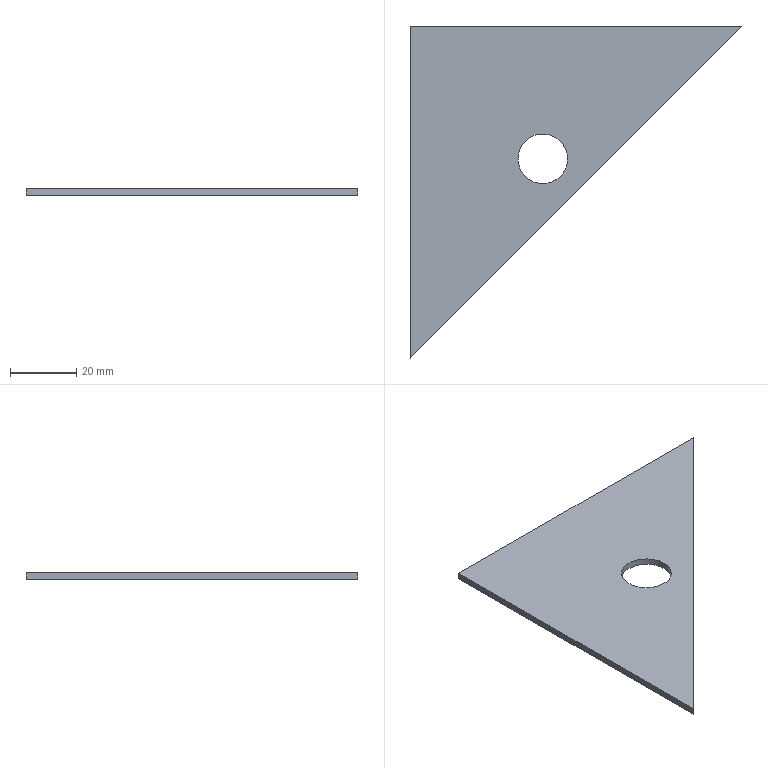Component | SolidWorks | GussetPlateAssembly-1_GussetPlate-1 | 1 solid | 7 faces | box 100 x 100 x 2 mm | volume 9647 mm3 | plane 5 | cylinder 2 | commonest cylinder face diameters 15 x2
STEP:
#1=CARTESIAN_POINT('',(-17.916,13.265,3.071));
#2=VERTEX_POINT('',#1);
#3=CARTESIAN_POINT('',(-17.326,13.265,3.071));
#4=VERTEX_POINT('',#3);
#5=CARTESIAN_POINT('',(-17.621,13.265,3.071));
#6=DIRECTION('',(0.,-0.,-1.));
#7=DIRECTION('',(1.,0.,0.));
#8=AXIS2_PLACEMENT_3D('',#5,#6,#7);
#9=CIRCLE('',#8,0.2953);
#10=EDGE_CURVE('',#2,#4,#9,.T.);
#11=ORIENTED_EDGE('',*,*,#10,.F.);
#12=CARTESIAN_POINT('',(-17.916,13.265,2.992));
#13=VERTEX_POINT('',#12);
#14=CARTESIAN_POINT('',(-17.916,13.265,3.071));
#15=DIRECTION('',(0.,-0.,-1.));
#16=VECTOR('',#15,39.37);
#17=LINE('',#14,#16);
#18=EDGE_CURVE('',#2,#13,#17,.T.);
#19=ORIENTED_EDGE('',*,*,#18,.T.);
#20=CARTESIAN_POINT('',(-17.326,13.265,2.992));
#21=VERTEX_POINT('',#20);
#22=CARTESIAN_POINT('',(-17.621,13.265,2.992));
#23=DIRECTION('',(0.,-0.,-1.));
#24=DIRECTION('',(1.,0.,0.));
#25=AXIS2_PLACEMENT_3D('',#22,#23,#24);
#26=CIRCLE('',#25,0.2953);
#27=EDGE_CURVE('',#13,#21,#26,.T.);
#28=ORIENTED_EDGE('',*,*,#27,.T.);
#29=CARTESIAN_POINT('',(-17.326,13.265,3.071));
#30=DIRECTION('',(0.,-0.,-1.));
#31=VECTOR('',#30,39.37);
#32=LINE('',#29,#31);
#33=EDGE_CURVE('',#4,#21,#32,.T.);
#34=ORIENTED_EDGE('',*,*,#33,.F.);
#35=EDGE_LOOP('',(#11,#19,#28,#34));
#36=FACE_OUTER_BOUND('',#35,.T.);
#37=CARTESIAN_POINT('',(-17.621,13.265,3.071));
#38=DIRECTION('',(0.,-0.,-1.));
#39=DIRECTION('',(1.,0.,0.));
#40=AXIS2_PLACEMENT_3D('',#37,#38,#39);
#41=CYLINDRICAL_SURFACE('',#40,0.2953);
#42=ADVANCED_FACE('',(#36),#41,.F.);
#43=CARTESIAN_POINT('',(-15.259,14.839,2.992));
#44=VERTEX_POINT('',#43);
#45=CARTESIAN_POINT('',(-19.196,10.902,2.992));
#46=VERTEX_POINT('',#45);
#47=CARTESIAN_POINT('',(-19.196,10.902,2.992));
#48=DIRECTION('',(-0.7071,-0.7071,-0.));
#49=VECTOR('',#48,39.37);
#50=LINE('',#47,#49);
#51=EDGE_CURVE('',#44,#46,#50,.T.);
#52=ORIENTED_EDGE('',*,*,#51,.F.);
#53=CARTESIAN_POINT('',(-15.259,14.839,3.071));
#54=VERTEX_POINT('',#53);
#55=CARTESIAN_POINT('',(-15.259,14.839,3.071));
#56=DIRECTION('',(0.,-0.,-1.));
#57=VECTOR('',#56,39.37);
#58=LINE('',#55,#57);
#59=EDGE_CURVE('',#54,#44,#58,.T.);
#60=ORIENTED_EDGE('',*,*,#59,.F.);
#61=CARTESIAN_POINT('',(-19.196,10.902,3.071));
#62=VERTEX_POINT('',#61);
#63=CARTESIAN_POINT('',(-19.196,10.902,3.071));
#64=DIRECTION('',(-0.7071,-0.7071,-0.));
#65=VECTOR('',#64,39.37);
#66=LINE('',#63,#65);
#67=EDGE_CURVE('',#54,#62,#66,.T.);
#68=ORIENTED_EDGE('',*,*,#67,.T.);
#69=CARTESIAN_POINT('',(-19.196,10.902,3.071));
#70=DIRECTION('',(0.,-0.,-1.));
#71=VECTOR('',#70,39.37);
#72=LINE('',#69,#71);
#73=EDGE_CURVE('',#62,#46,#72,.T.);
#74=ORIENTED_EDGE('',*,*,#73,.T.);
#75=EDGE_LOOP('',(#52,#60,#68,#74));
#76=FACE_OUTER_BOUND('',#75,.T.);
#77=CARTESIAN_POINT('',(-19.196,10.902,3.071));
#78=DIRECTION('',(0.7071,-0.7071,0.));
#79=DIRECTION('',(-0.7071,-0.7071,-0.));
#80=AXIS2_PLACEMENT_3D('',#77,#78,#79);
#81=PLANE('',#80);
#82=ADVANCED_FACE('',(#76),#81,.T.);
#83=CARTESIAN_POINT('',(-19.196,14.839,2.992));
#84=VERTEX_POINT('',#83);
#85=CARTESIAN_POINT('',(-19.196,14.839,2.992));
#86=DIRECTION('',(1.,0.,0.));
#87=VECTOR('',#86,39.37);
#88=LINE('',#85,#87);
#89=EDGE_CURVE('',#84,#44,#88,.T.);
#90=ORIENTED_EDGE('',*,*,#89,.F.);
#91=CARTESIAN_POINT('',(-19.196,14.839,3.071));
#92=VERTEX_POINT('',#91);
#93=CARTESIAN_POINT('',(-19.196,14.839,3.071));
#94=DIRECTION('',(0.,-0.,-1.));
#95=VECTOR('',#94,39.37);
#96=LINE('',#93,#95);
#97=EDGE_CURVE('',#92,#84,#96,.T.);
#98=ORIENTED_EDGE('',*,*,#97,.F.);
#99=CARTESIAN_POINT('',(-19.196,14.839,3.071));
#100=DIRECTION('',(1.,0.,0.));
#101=VECTOR('',#100,39.37);
#102=LINE('',#99,#101);
#103=EDGE_CURVE('',#92,#54,#102,.T.);
#104=ORIENTED_EDGE('',*,*,#103,.T.);
#105=ORIENTED_EDGE('',*,*,#59,.T.);
#106=EDGE_LOOP('',(#90,#98,#104,#105));
#107=FACE_OUTER_BOUND('',#106,.T.);
#108=CARTESIAN_POINT('',(-19.196,14.839,3.071));
#109=DIRECTION('',(-0.,1.,-0.));
#110=DIRECTION('',(-0.,0.,1.));
#111=AXIS2_PLACEMENT_3D('',#108,#109,#110);
#112=PLANE('',#111);
#113=ADVANCED_FACE('',(#107),#112,.T.);
#114=CARTESIAN_POINT('',(-19.196,10.902,2.992));
#115=DIRECTION('',(-0.,1.,-0.));
#116=VECTOR('',#115,39.37);
#117=LINE('',#114,#116);
#118=EDGE_CURVE('',#46,#84,#117,.T.);
#119=ORIENTED_EDGE('',*,*,#118,.F.);
#120=ORIENTED_EDGE('',*,*,#73,.F.);
#121=CARTESIAN_POINT('',(-19.196,10.902,3.071));
#122=DIRECTION('',(-0.,1.,-0.));
#123=VECTOR('',#122,39.37);
#124=LINE('',#121,#123);
#125=EDGE_CURVE('',#62,#92,#124,.T.);
#126=ORIENTED_EDGE('',*,*,#125,.T.);
#127=ORIENTED_EDGE('',*,*,#97,.T.);
#128=EDGE_LOOP('',(#119,#120,#126,#127));
#129=FACE_OUTER_BOUND('',#128,.T.);
#130=CARTESIAN_POINT('',(-19.196,10.902,3.071));
#131=DIRECTION('',(-1.,-0.,-0.));
#132=DIRECTION('',(-0.,1.,-0.));
#133=AXIS2_PLACEMENT_3D('',#130,#131,#132);
#134=PLANE('',#133);
#135=ADVANCED_FACE('',(#129),#134,.T.);
#136=CARTESIAN_POINT('',(-17.621,13.265,3.071));
#137=DIRECTION('',(0.,-0.,-1.));
#138=DIRECTION('',(1.,0.,0.));
#139=AXIS2_PLACEMENT_3D('',#136,#137,#138);
#140=CIRCLE('',#139,0.2953);
#141=EDGE_CURVE('',#4,#2,#140,.T.);
#142=ORIENTED_EDGE('',*,*,#141,.T.);
#143=ORIENTED_EDGE('',*,*,#10,.T.);
#144=EDGE_LOOP('',(#142,#143));
#145=FACE_BOUND('',#144,.T.);
#146=ORIENTED_EDGE('',*,*,#67,.F.);
#147=ORIENTED_EDGE('',*,*,#103,.F.);
#148=ORIENTED_EDGE('',*,*,#125,.F.);
#149=EDGE_LOOP('',(#146,#147,#148));
#150=FACE_OUTER_BOUND('',#149,.T.);
#151=CARTESIAN_POINT('',(-15.259,14.839,3.071));
#152=DIRECTION('',(0.,-0.,-1.));
#153=DIRECTION('',(1.,0.,0.));
#154=AXIS2_PLACEMENT_3D('',#151,#152,#153);
#155=PLANE('',#154);
#156=ADVANCED_FACE('',(#145,#150),#155,.F.);
#157=CARTESIAN_POINT('',(-17.621,13.265,2.992));
#158=DIRECTION('',(0.,-0.,-1.));
#159=DIRECTION('',(1.,0.,0.));
#160=AXIS2_PLACEMENT_3D('',#157,#158,#159);
#161=CIRCLE('',#160,0.2953);
#162=EDGE_CURVE('',#21,#13,#161,.T.);
#163=ORIENTED_EDGE('',*,*,#162,.F.);
#164=ORIENTED_EDGE('',*,*,#27,.F.);
#165=EDGE_LOOP('',(#163,#164));
#166=FACE_BOUND('',#165,.T.);
#167=ORIENTED_EDGE('',*,*,#51,.T.);
#168=ORIENTED_EDGE('',*,*,#118,.T.);
#169=ORIENTED_EDGE('',*,*,#89,.T.);
#170=EDGE_LOOP('',(#167,#168,#169));
#171=FACE_OUTER_BOUND('',#170,.T.);
#172=CARTESIAN_POINT('',(-15.259,14.839,2.992));
#173=DIRECTION('',(0.,-0.,-1.));
#174=DIRECTION('',(1.,0.,0.));
#175=AXIS2_PLACEMENT_3D('',#172,#173,#174);
#176=PLANE('',#175);
#177=ADVANCED_FACE('',(#166,#171),#176,.T.);
#178=ORIENTED_EDGE('',*,*,#18,.F.);
#179=ORIENTED_EDGE('',*,*,#141,.F.);
#180=ORIENTED_EDGE('',*,*,#33,.T.);
#181=ORIENTED_EDGE('',*,*,#162,.T.);
#182=EDGE_LOOP('',(#178,#179,#180,#181));
#183=FACE_OUTER_BOUND('',#182,.T.);
#184=CARTESIAN_POINT('',(-17.621,13.265,3.071));
#185=DIRECTION('',(0.,-0.,-1.));
#186=DIRECTION('',(1.,0.,0.));
#187=AXIS2_PLACEMENT_3D('',#184,#185,#186);
#188=CYLINDRICAL_SURFACE('',#187,0.2953);
#189=ADVANCED_FACE('',(#183),#188,.F.);
#190=CLOSED_SHELL('',(#42,#82,#113,#135,#156,#177,#189));
#191=MANIFOLD_SOLID_BREP('',#190);
#192=CARTESIAN_POINT('',(0.,0.,0.));
#193=DIRECTION('',(0.,0.,1.));
#194=DIRECTION('',(1.,0.,0.));
#195=AXIS2_PLACEMENT_3D('',#192,#193,#194);
#196=(LENGTH_UNIT()NAMED_UNIT(*)SI_UNIT($,.METRE.));
#197=LENGTH_MEASURE_WITH_UNIT(LENGTH_MEASURE(0.0254),#196);
#198=DIMENSIONAL_EXPONENTS(1.,0.,0.,0.,0.,0.,0.);
#199=(CONVERSION_BASED_UNIT('',#197)LENGTH_UNIT()NAMED_UNIT(#198));
#200=UNCERTAINTY_MEASURE_WITH_UNIT(LENGTH_MEASURE(0.00001),#199,'','');
#201=(NAMED_UNIT(*)PLANE_ANGLE_UNIT()SI_UNIT($,.RADIAN.));
#202=(NAMED_UNIT(*)SI_UNIT($,.STERADIAN.)SOLID_ANGLE_UNIT());
#203=(GEOMETRIC_REPRESENTATION_CONTEXT(3)GLOBAL_UNCERTAINTY_ASSIGNED_CONTEXT((#200))GLOBAL_UNIT_ASSIGNED_CONTEXT((#199,#201,#202))REPRESENTATION_CONTEXT('',''));
#204=ADVANCED_BREP_SHAPE_REPRESENTATION('',(#191,#195),#203);
#205=COLOUR_RGB('',0.7922,0.8196,0.9333);
#206=FILL_AREA_STYLE_COLOUR('',#205);
#207=FILL_AREA_STYLE('',(#206));
#208=SURFACE_STYLE_FILL_AREA(#207);
#209=SURFACE_SIDE_STYLE('',(#208));
#210=SURFACE_STYLE_USAGE(.BOTH.,#209);
#211=PRESENTATION_STYLE_ASSIGNMENT((#210));
#212=STYLED_ITEM('',(#211),#191);
#213=PRESENTATION_LAYER_ASSIGNMENT('','',(#212));
#214=(LENGTH_UNIT()NAMED_UNIT(*)SI_UNIT($,.METRE.));
#215=LENGTH_MEASURE_WITH_UNIT(LENGTH_MEASURE(0.0254),#214);
#216=DIMENSIONAL_EXPONENTS(1.,0.,0.,0.,0.,0.,0.);
#217=(CONVERSION_BASED_UNIT('',#215)LENGTH_UNIT()NAMED_UNIT(#216));
#218=UNCERTAINTY_MEASURE_WITH_UNIT(LENGTH_MEASURE(0.00001),#217,'','');
#219=(NAMED_UNIT(*)PLANE_ANGLE_UNIT()SI_UNIT($,.RADIAN.));
#220=(NAMED_UNIT(*)SI_UNIT($,.STERADIAN.)SOLID_ANGLE_UNIT());
#221=(GEOMETRIC_REPRESENTATION_CONTEXT(3)GLOBAL_UNCERTAINTY_ASSIGNED_CONTEXT((#218))GLOBAL_UNIT_ASSIGNED_CONTEXT((#217,#219,#220))REPRESENTATION_CONTEXT('',''));
#222=MECHANICAL_DESIGN_GEOMETRIC_PRESENTATION_REPRESENTATION('',(#212),#221);